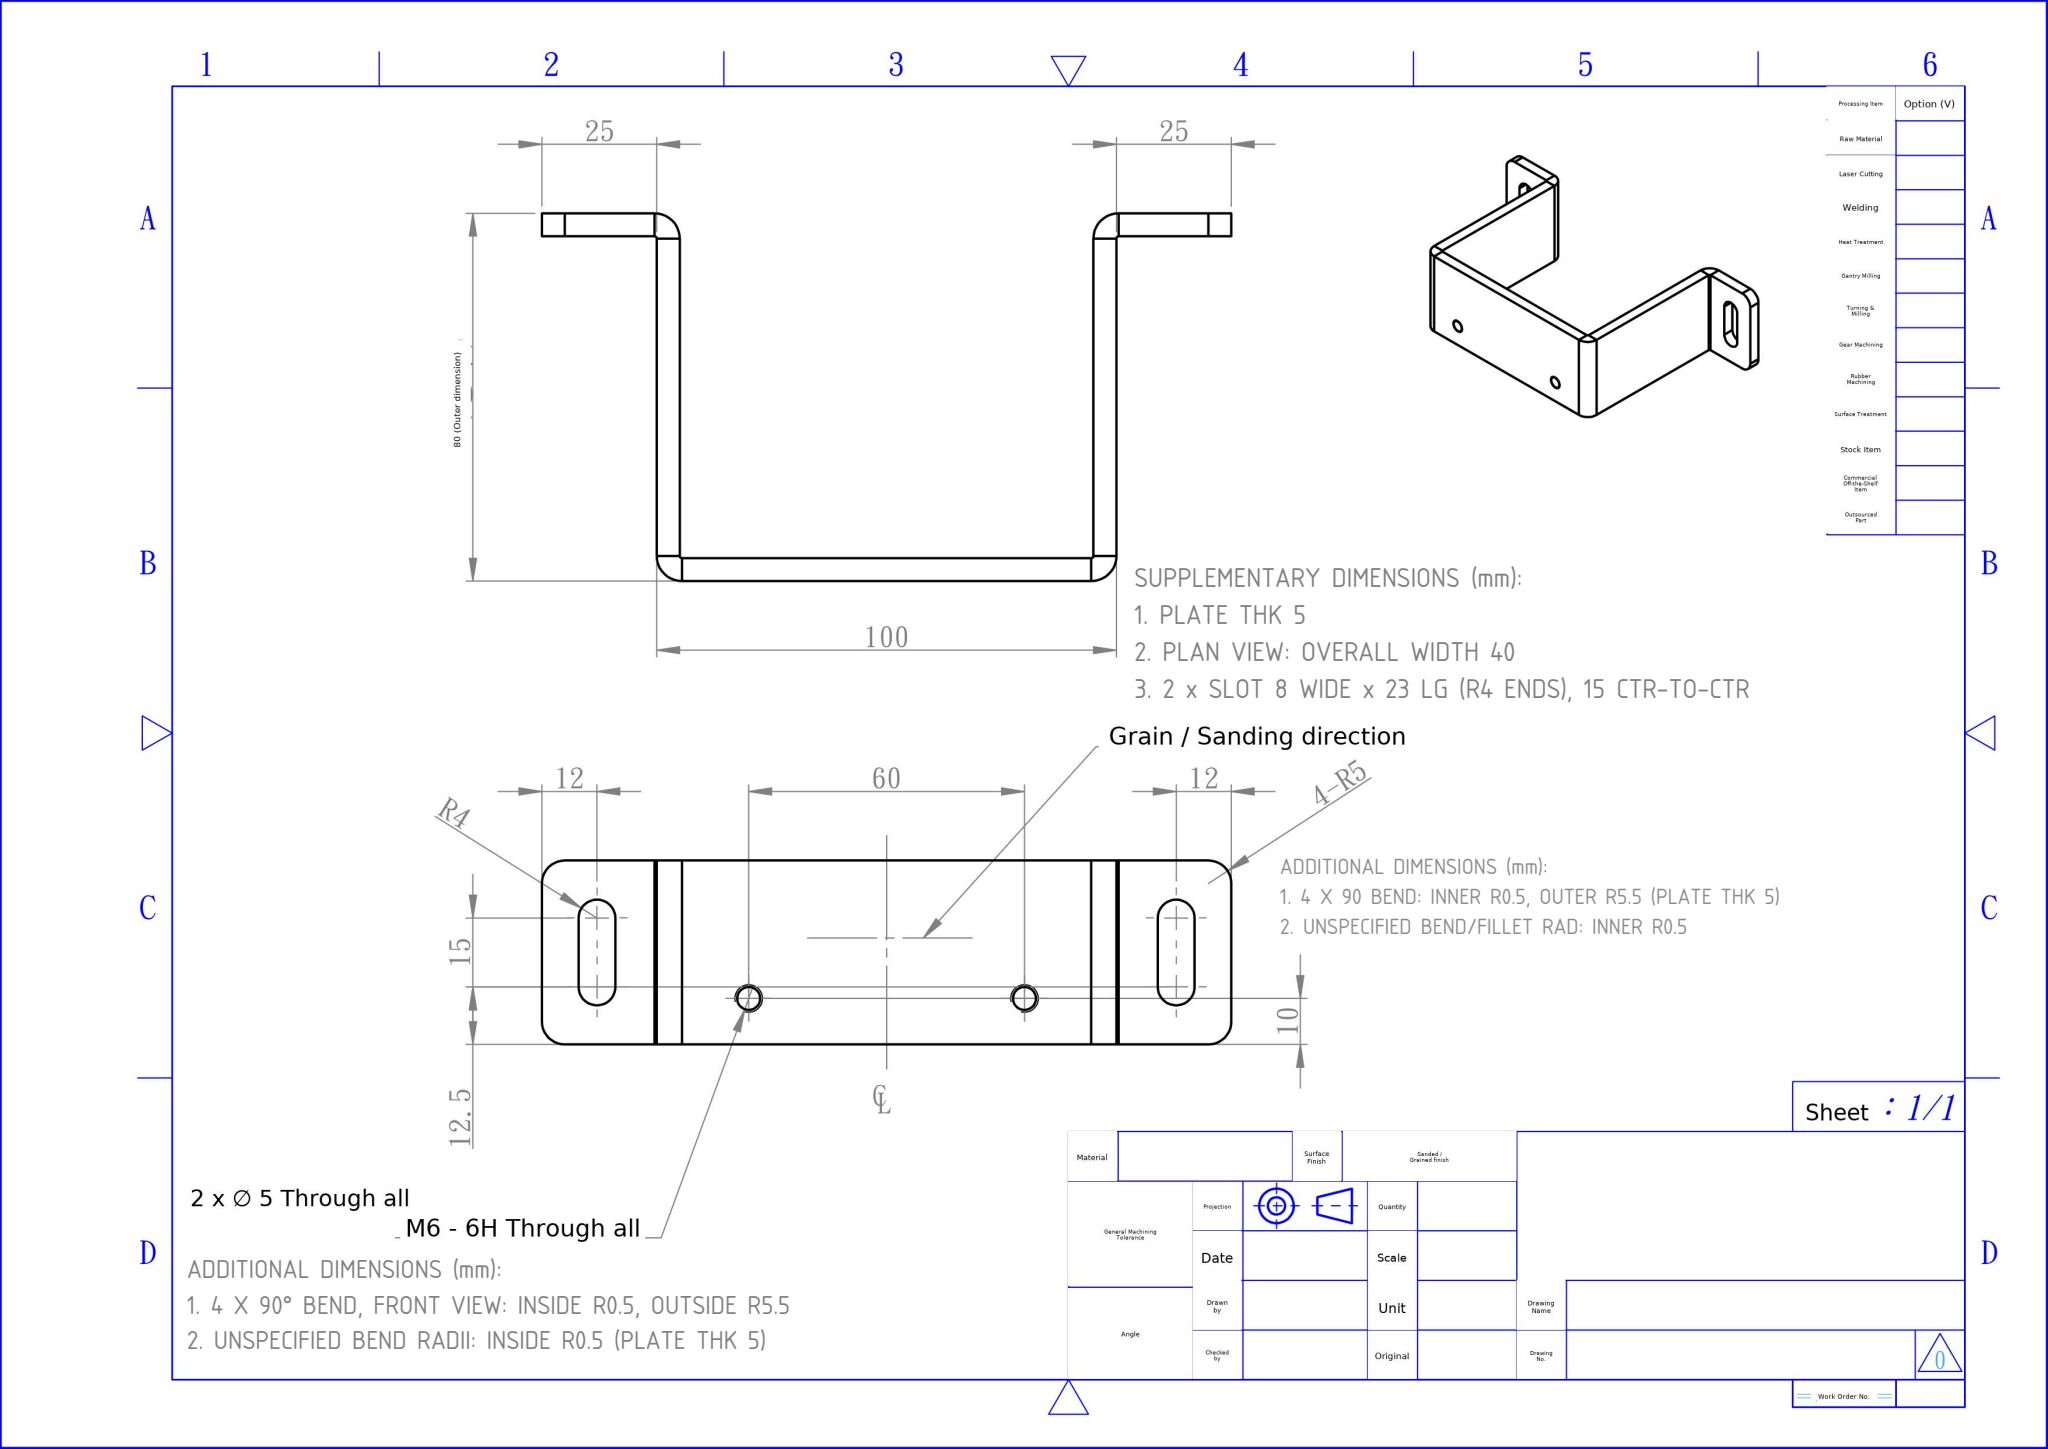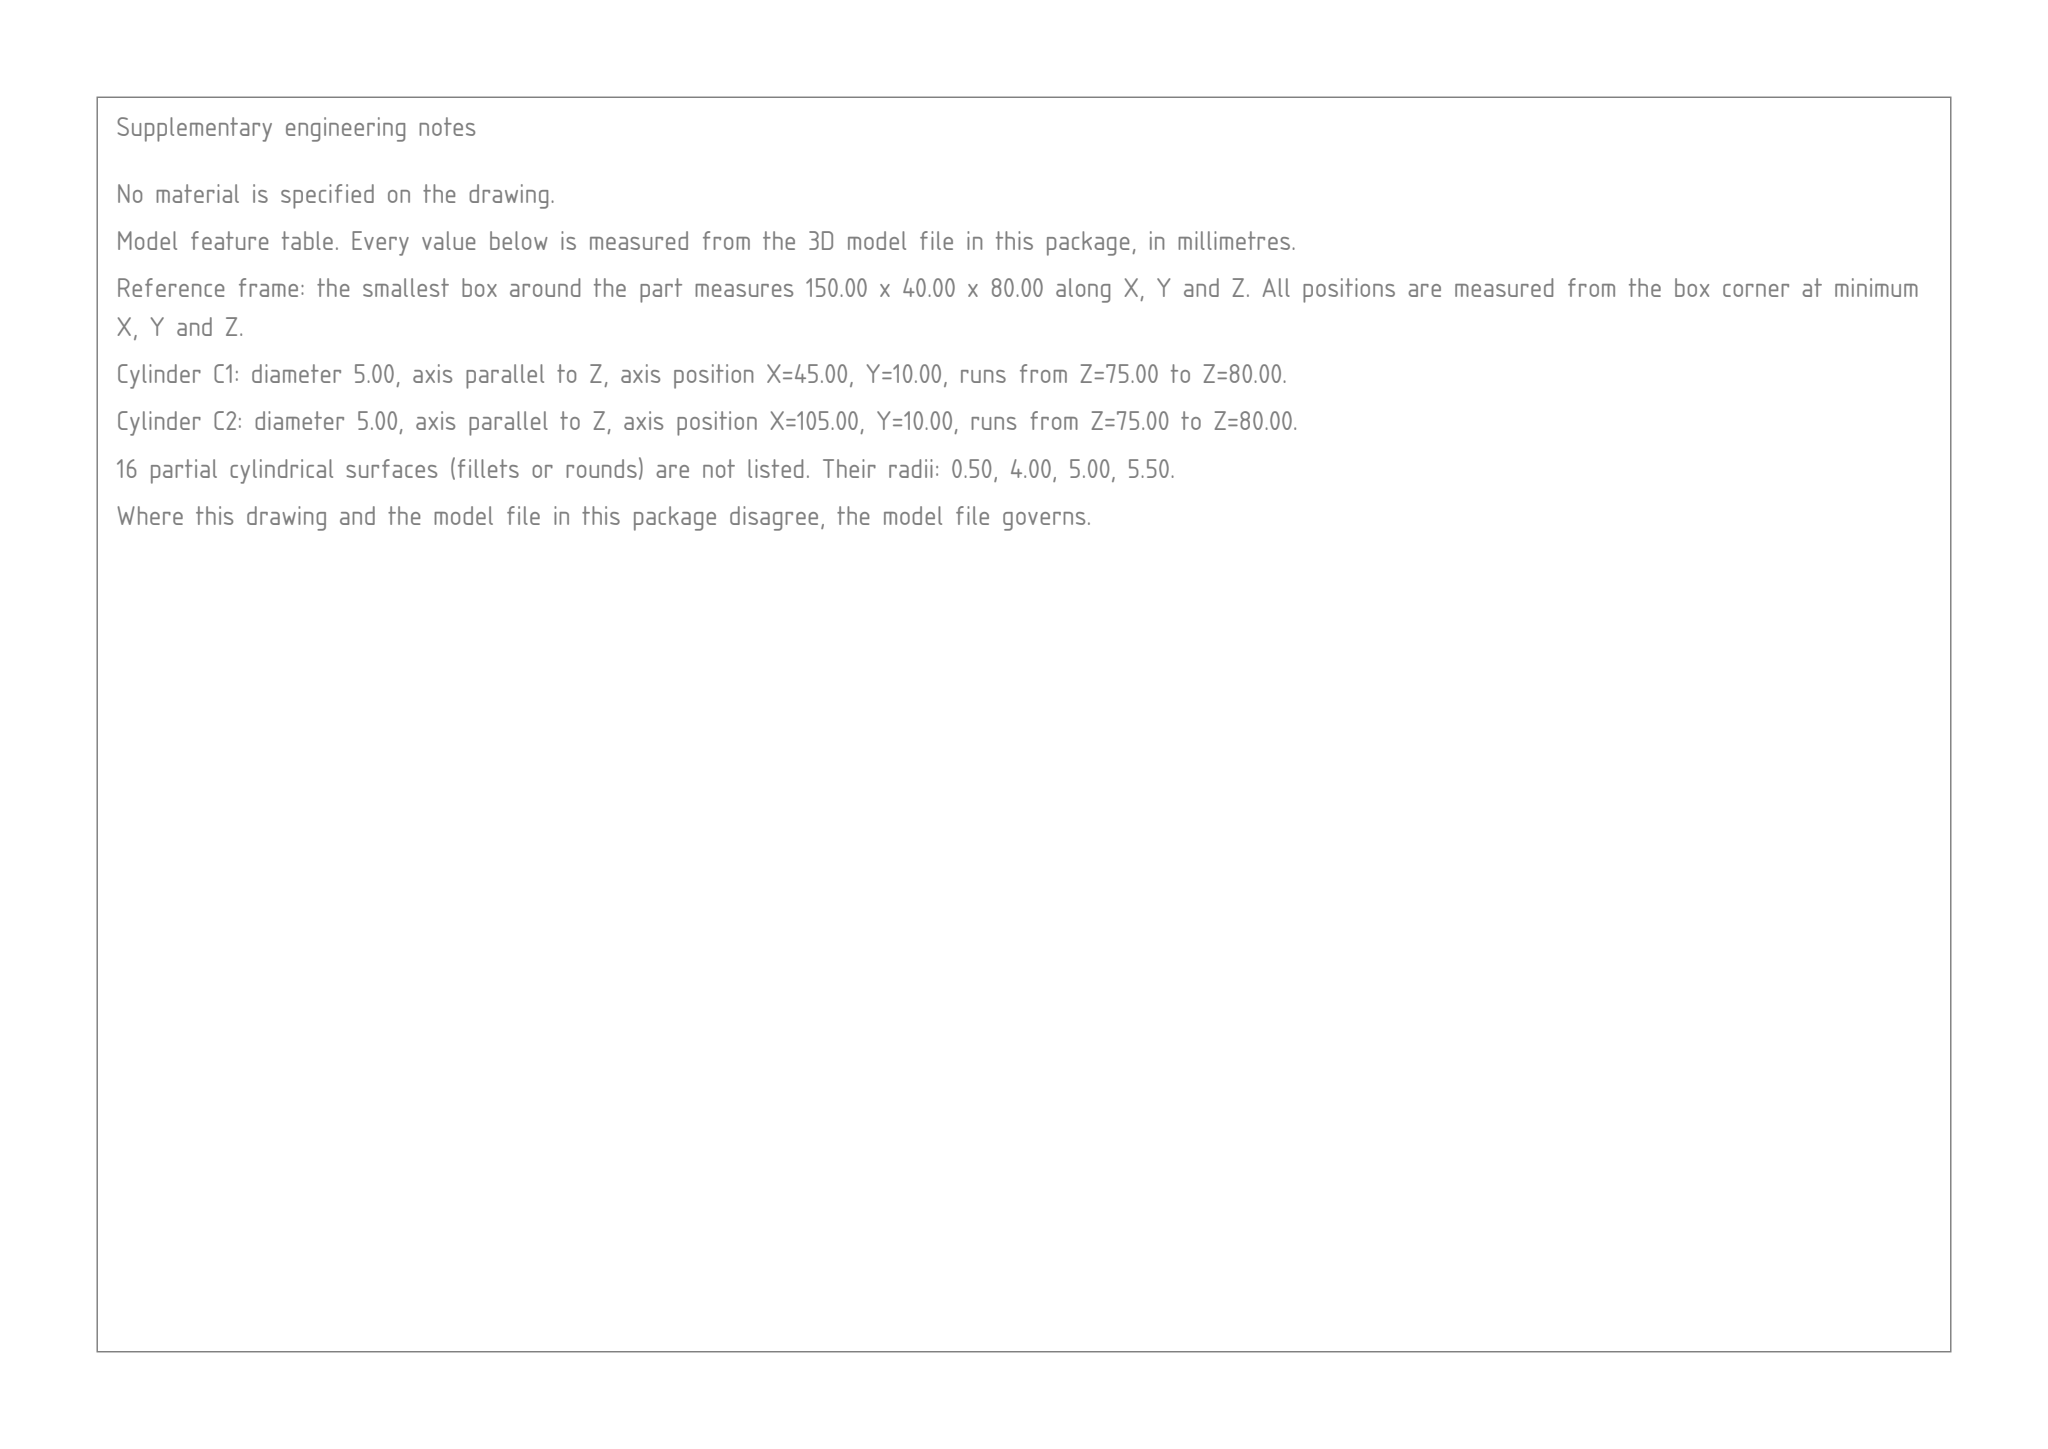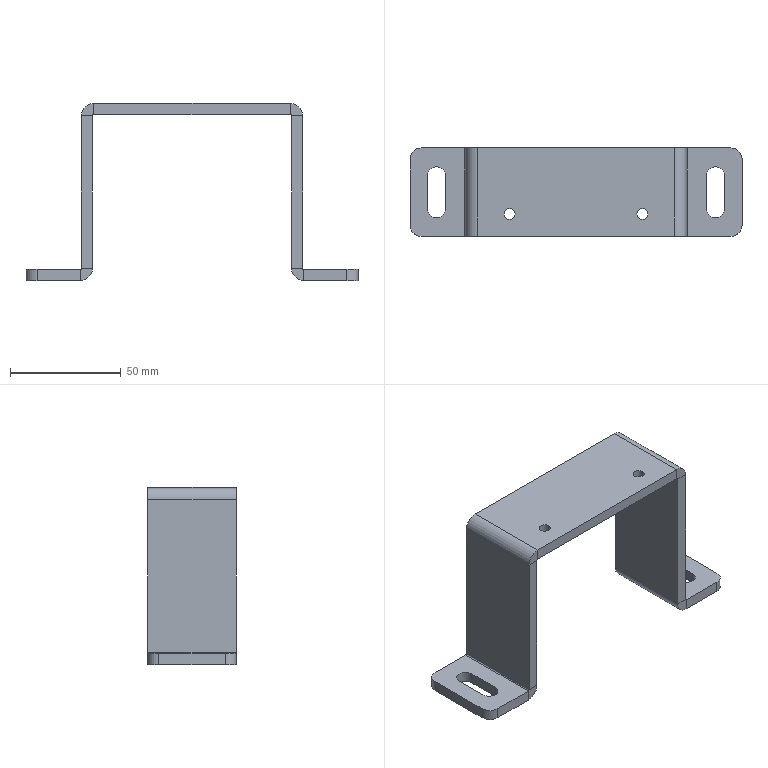Part | SolidWorks | mm | 1 solid | 54 faces | box 150 x 40 x 80 mm | volume 56964 mm3 | plane 34 | cylinder 20 | commonest cylinder face diameters 5 x4 11 x4 1 x4 8 x4 10 x4